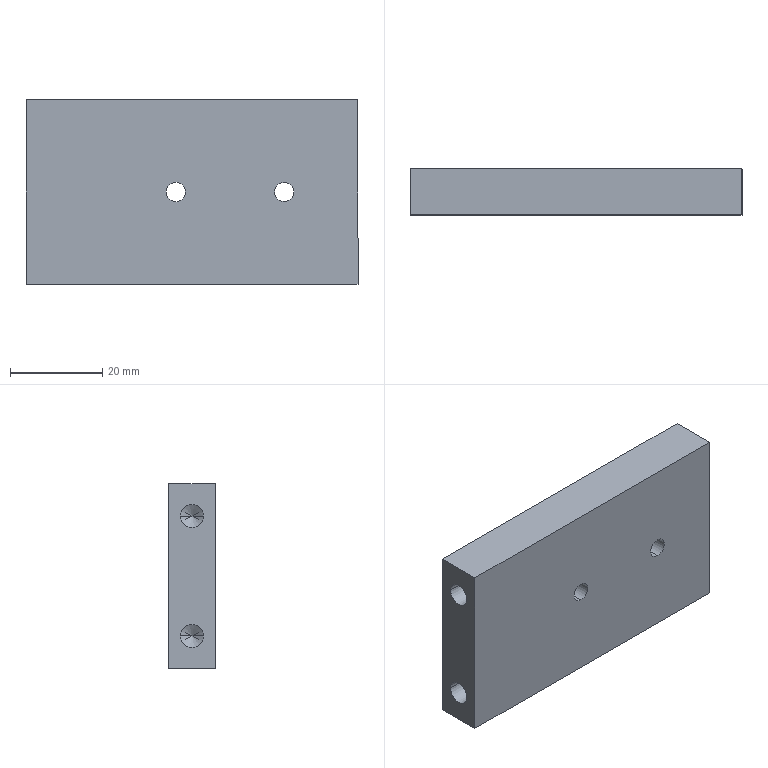Component | SolidWorks | SL021-102-4074.SL4PRT-1 | 1 solid | 18 faces | box 72 x 10 x 40 mm | volume 27718 mm3 | cylinder 8 | plane 6 | cone 4 | commonest cylinder face diameters 4.2 x4 5 x4 | material AL6061
build123d program:
from build123d import *

# Parameters (mm, degrees)
SKETCH1_W             = 40
SKETCH1_H             = 72
BOSS_EXTRUDE1_DEPTH   = 5
M6_TAPPED_HOLE1_D     = 5
M6_TAPPED_HOLE1_DEPTH = 20
M6_TAPPED_HOLE1_TIP   = 1.502
M5_TAPPED_HOLE1_D     = 4.2


with BuildPart() as part:
    # Sketch1 → Boss-Extrude1 (new, symmetric)
    with BuildSketch(Plane.XY):
        Rectangle(SKETCH1_W, SKETCH1_H)
    extrude(amount=BOSS_EXTRUDE1_DEPTH, both=True)

    # M6 Tapped Hole1
    with Locations(Plane(origin=(0, -36, -55), x_dir=(1, 0, 0), z_dir=(0, -1, 0))):
        with Locations((-13, 55), (13, 55)):
            Hole(M6_TAPPED_HOLE1_D / 2, depth=M6_TAPPED_HOLE1_DEPTH)
            with Locations((0, 0, -(M6_TAPPED_HOLE1_DEPTH + M6_TAPPED_HOLE1_TIP / 2))):  # 118° drill point
                Cone(0, M6_TAPPED_HOLE1_D / 2, M6_TAPPED_HOLE1_TIP, mode=Mode.SUBTRACT)

    # M5 Tapped Hole1 (through all)
    with Locations(Plane.XY.offset(5)):
        with Locations((0, 20), (0, -3.5)):
            Hole(M5_TAPPED_HOLE1_D / 2)


solid = part.part

# Placed as in the assembly
solid = solid.moved(Location((71.837, 179.501, -198.378), (90, 0, -90)))
STEP:
#1=COLOUR_RGB('',0.7922,0.8196,0.9333);
#2=FILL_AREA_STYLE_COLOUR('',#1);
#3=FILL_AREA_STYLE('',(#2));
#4=SURFACE_STYLE_FILL_AREA(#3);
#5=SURFACE_SIDE_STYLE('',(#4));
#6=SURFACE_STYLE_USAGE(.BOTH.,#5);
#7=PRESENTATION_STYLE_ASSIGNMENT((#6));
#8=CARTESIAN_POINT('',(3.616,6.87,-7.893));
#9=VERTEX_POINT('',#8);
#10=CARTESIAN_POINT('',(3.616,6.87,-7.727));
#11=VERTEX_POINT('',#10);
#12=CARTESIAN_POINT('',(3.616,6.87,-7.81));
#13=DIRECTION('',(0.,1.,0.));
#14=DIRECTION('',(0.,0.,1.));
#15=AXIS2_PLACEMENT_3D('',#12,#13,#14);
#16=CIRCLE('',#15,0.08268);
#17=EDGE_CURVE('',#9,#11,#16,.T.);
#18=ORIENTED_EDGE('',*,*,#17,.F.);
#19=CARTESIAN_POINT('',(3.616,7.264,-7.893));
#20=VERTEX_POINT('',#19);
#21=CARTESIAN_POINT('',(3.616,7.264,-7.893));
#22=DIRECTION('',(0.,1.,0.));
#23=VECTOR('',#22,39.37);
#24=LINE('',#21,#23);
#25=EDGE_CURVE('',#9,#20,#24,.T.);
#26=ORIENTED_EDGE('',*,*,#25,.T.);
#27=CARTESIAN_POINT('',(3.616,7.264,-7.727));
#28=VERTEX_POINT('',#27);
#29=CARTESIAN_POINT('',(3.616,7.264,-7.81));
#30=DIRECTION('',(0.,1.,0.));
#31=DIRECTION('',(0.,0.,1.));
#32=AXIS2_PLACEMENT_3D('',#29,#30,#31);
#33=CIRCLE('',#32,0.08268);
#34=EDGE_CURVE('',#20,#28,#33,.T.);
#35=ORIENTED_EDGE('',*,*,#34,.T.);
#36=CARTESIAN_POINT('',(3.616,7.264,-7.727));
#37=DIRECTION('',(0.,1.,0.));
#38=VECTOR('',#37,39.37);
#39=LINE('',#36,#38);
#40=EDGE_CURVE('',#11,#28,#39,.T.);
#41=ORIENTED_EDGE('',*,*,#40,.F.);
#42=EDGE_LOOP('',(#18,#26,#35,#41));
#43=FACE_OUTER_BOUND('',#42,.T.);
#44=CARTESIAN_POINT('',(3.616,7.264,-7.81));
#45=DIRECTION('',(0.,1.,0.));
#46=DIRECTION('',(0.,0.,1.));
#47=AXIS2_PLACEMENT_3D('',#44,#45,#46);
#48=CYLINDRICAL_SURFACE('',#47,0.08268);
#49=ADVANCED_FACE('',(#43),#48,.F.);
#50=CARTESIAN_POINT('',(2.69,6.87,-7.893));
#51=VERTEX_POINT('',#50);
#52=CARTESIAN_POINT('',(2.69,6.87,-7.727));
#53=VERTEX_POINT('',#52);
#54=CARTESIAN_POINT('',(2.69,6.87,-7.81));
#55=DIRECTION('',(0.,1.,0.));
#56=DIRECTION('',(0.,0.,1.));
#57=AXIS2_PLACEMENT_3D('',#54,#55,#56);
#58=CIRCLE('',#57,0.08268);
#59=EDGE_CURVE('',#51,#53,#58,.T.);
#60=ORIENTED_EDGE('',*,*,#59,.F.);
#61=CARTESIAN_POINT('',(2.69,7.264,-7.893));
#62=VERTEX_POINT('',#61);
#63=CARTESIAN_POINT('',(2.69,7.264,-7.893));
#64=DIRECTION('',(0.,1.,0.));
#65=VECTOR('',#64,39.37);
#66=LINE('',#63,#65);
#67=EDGE_CURVE('',#51,#62,#66,.T.);
#68=ORIENTED_EDGE('',*,*,#67,.T.);
#69=CARTESIAN_POINT('',(2.69,7.264,-7.727));
#70=VERTEX_POINT('',#69);
#71=CARTESIAN_POINT('',(2.69,7.264,-7.81));
#72=DIRECTION('',(0.,1.,0.));
#73=DIRECTION('',(0.,0.,1.));
#74=AXIS2_PLACEMENT_3D('',#71,#72,#73);
#75=CIRCLE('',#74,0.08268);
#76=EDGE_CURVE('',#62,#70,#75,.T.);
#77=ORIENTED_EDGE('',*,*,#76,.T.);
#78=CARTESIAN_POINT('',(2.69,7.264,-7.727));
#79=DIRECTION('',(0.,1.,0.));
#80=VECTOR('',#79,39.37);
#81=LINE('',#78,#80);
#82=EDGE_CURVE('',#53,#70,#81,.T.);
#83=ORIENTED_EDGE('',*,*,#82,.F.);
#84=EDGE_LOOP('',(#60,#68,#77,#83));
#85=FACE_OUTER_BOUND('',#84,.T.);
#86=CARTESIAN_POINT('',(2.69,7.264,-7.81));
#87=DIRECTION('',(0.,1.,0.));
#88=DIRECTION('',(0.,0.,1.));
#89=AXIS2_PLACEMENT_3D('',#86,#87,#88);
#90=CYLINDRICAL_SURFACE('',#89,0.08268);
#91=ADVANCED_FACE('',(#85),#90,.F.);
#92=CARTESIAN_POINT('',(2.198,7.165,-8.322));
#93=VERTEX_POINT('',#92);
#94=CARTESIAN_POINT('',(2.198,6.969,-8.322));
#95=VERTEX_POINT('',#94);
#96=CARTESIAN_POINT('',(2.198,7.067,-8.322));
#97=DIRECTION('',(-1.,0.,-0.));
#98=DIRECTION('',(0.,-1.,0.));
#99=AXIS2_PLACEMENT_3D('',#96,#97,#98);
#100=CIRCLE('',#99,0.09843);
#101=EDGE_CURVE('',#93,#95,#100,.T.);
#102=ORIENTED_EDGE('',*,*,#101,.F.);
#103=CARTESIAN_POINT('',(1.411,7.165,-8.322));
#104=VERTEX_POINT('',#103);
#105=CARTESIAN_POINT('',(1.411,7.165,-8.322));
#106=DIRECTION('',(-1.,0.,-0.));
#107=VECTOR('',#106,39.37);
#108=LINE('',#105,#107);
#109=EDGE_CURVE('',#93,#104,#108,.T.);
#110=ORIENTED_EDGE('',*,*,#109,.T.);
#111=CARTESIAN_POINT('',(1.411,6.969,-8.322));
#112=VERTEX_POINT('',#111);
#113=CARTESIAN_POINT('',(1.411,7.067,-8.322));
#114=DIRECTION('',(-1.,0.,-0.));
#115=DIRECTION('',(0.,-1.,0.));
#116=AXIS2_PLACEMENT_3D('',#113,#114,#115);
#117=CIRCLE('',#116,0.09843);
#118=EDGE_CURVE('',#104,#112,#117,.T.);
#119=ORIENTED_EDGE('',*,*,#118,.T.);
#120=CARTESIAN_POINT('',(1.411,6.969,-8.322));
#121=DIRECTION('',(-1.,0.,-0.));
#122=VECTOR('',#121,39.37);
#123=LINE('',#120,#122);
#124=EDGE_CURVE('',#95,#112,#123,.T.);
#125=ORIENTED_EDGE('',*,*,#124,.F.);
#126=EDGE_LOOP('',(#102,#110,#119,#125));
#127=FACE_OUTER_BOUND('',#126,.T.);
#128=CARTESIAN_POINT('',(1.411,7.067,-8.322));
#129=DIRECTION('',(-1.,0.,-0.));
#130=DIRECTION('',(0.,-1.,0.));
#131=AXIS2_PLACEMENT_3D('',#128,#129,#130);
#132=CYLINDRICAL_SURFACE('',#131,0.09843);
#133=ADVANCED_FACE('',(#127),#132,.F.);
#134=CARTESIAN_POINT('',(2.257,7.067,-8.322));
#135=VERTEX_POINT('',#134);
#136=CARTESIAN_POINT('',(2.198,6.969,-8.322));
#137=DIRECTION('',(-0.515,-0.8572,-0.));
#138=VECTOR('',#137,39.37);
#139=LINE('',#136,#138);
#140=EDGE_CURVE('',#135,#95,#139,.T.);
#141=ORIENTED_EDGE('',*,*,#140,.F.);
#142=CARTESIAN_POINT('',(2.198,7.165,-8.322));
#143=DIRECTION('',(-0.515,0.8572,0.));
#144=VECTOR('',#143,39.37);
#145=LINE('',#142,#144);
#146=EDGE_CURVE('',#135,#93,#145,.T.);
#147=ORIENTED_EDGE('',*,*,#146,.T.);
#148=ORIENTED_EDGE('',*,*,#101,.T.);
#149=EDGE_LOOP('',(#141,#147,#148));
#150=FACE_OUTER_BOUND('',#149,.T.);
#151=CARTESIAN_POINT('',(2.198,7.067,-8.322));
#152=DIRECTION('',(-1.,0.,-0.));
#153=DIRECTION('',(0.,-1.,0.));
#154=AXIS2_PLACEMENT_3D('',#151,#152,#153);
#155=CONICAL_SURFACE('',#154,0.09843,1.03);
#156=ADVANCED_FACE('',(#150),#155,.F.);
#157=CARTESIAN_POINT('',(2.198,7.165,-7.298));
#158=VERTEX_POINT('',#157);
#159=CARTESIAN_POINT('',(2.198,6.969,-7.298));
#160=VERTEX_POINT('',#159);
#161=CARTESIAN_POINT('',(2.198,7.067,-7.298));
#162=DIRECTION('',(-1.,0.,-0.));
#163=DIRECTION('',(0.,-1.,0.));
#164=AXIS2_PLACEMENT_3D('',#161,#162,#163);
#165=CIRCLE('',#164,0.09843);
#166=EDGE_CURVE('',#158,#160,#165,.T.);
#167=ORIENTED_EDGE('',*,*,#166,.F.);
#168=CARTESIAN_POINT('',(1.411,7.165,-7.298));
#169=VERTEX_POINT('',#168);
#170=CARTESIAN_POINT('',(1.411,7.165,-7.298));
#171=DIRECTION('',(-1.,0.,-0.));
#172=VECTOR('',#171,39.37);
#173=LINE('',#170,#172);
#174=EDGE_CURVE('',#158,#169,#173,.T.);
#175=ORIENTED_EDGE('',*,*,#174,.T.);
#176=CARTESIAN_POINT('',(1.411,6.969,-7.298));
#177=VERTEX_POINT('',#176);
#178=CARTESIAN_POINT('',(1.411,7.067,-7.298));
#179=DIRECTION('',(-1.,0.,-0.));
#180=DIRECTION('',(0.,-1.,0.));
#181=AXIS2_PLACEMENT_3D('',#178,#179,#180);
#182=CIRCLE('',#181,0.09843);
#183=EDGE_CURVE('',#169,#177,#182,.T.);
#184=ORIENTED_EDGE('',*,*,#183,.T.);
#185=CARTESIAN_POINT('',(1.411,6.969,-7.298));
#186=DIRECTION('',(-1.,0.,-0.));
#187=VECTOR('',#186,39.37);
#188=LINE('',#185,#187);
#189=EDGE_CURVE('',#160,#177,#188,.T.);
#190=ORIENTED_EDGE('',*,*,#189,.F.);
#191=EDGE_LOOP('',(#167,#175,#184,#190));
#192=FACE_OUTER_BOUND('',#191,.T.);
#193=CARTESIAN_POINT('',(1.411,7.067,-7.298));
#194=DIRECTION('',(-1.,0.,-0.));
#195=DIRECTION('',(0.,-1.,0.));
#196=AXIS2_PLACEMENT_3D('',#193,#194,#195);
#197=CYLINDRICAL_SURFACE('',#196,0.09843);
#198=ADVANCED_FACE('',(#192),#197,.F.);
#199=CARTESIAN_POINT('',(2.257,7.067,-7.298));
#200=VERTEX_POINT('',#199);
#201=CARTESIAN_POINT('',(2.198,6.969,-7.298));
#202=DIRECTION('',(-0.515,-0.8572,-0.));
#203=VECTOR('',#202,39.37);
#204=LINE('',#201,#203);
#205=EDGE_CURVE('',#200,#160,#204,.T.);
#206=ORIENTED_EDGE('',*,*,#205,.F.);
#207=CARTESIAN_POINT('',(2.198,7.165,-7.298));
#208=DIRECTION('',(-0.515,0.8572,0.));
#209=VECTOR('',#208,39.37);
#210=LINE('',#207,#209);
#211=EDGE_CURVE('',#200,#158,#210,.T.);
#212=ORIENTED_EDGE('',*,*,#211,.T.);
#213=ORIENTED_EDGE('',*,*,#166,.T.);
#214=EDGE_LOOP('',(#206,#212,#213));
#215=FACE_OUTER_BOUND('',#214,.T.);
#216=CARTESIAN_POINT('',(2.198,7.067,-7.298));
#217=DIRECTION('',(-1.,0.,-0.));
#218=DIRECTION('',(0.,-1.,0.));
#219=AXIS2_PLACEMENT_3D('',#216,#217,#218);
#220=CONICAL_SURFACE('',#219,0.09843,1.03);
#221=ADVANCED_FACE('',(#215),#220,.F.);
#222=CARTESIAN_POINT('',(1.411,6.87,-7.023));
#223=VERTEX_POINT('',#222);
#224=CARTESIAN_POINT('',(4.246,6.87,-7.023));
#225=VERTEX_POINT('',#224);
#226=CARTESIAN_POINT('',(1.411,6.87,-7.023));
#227=DIRECTION('',(1.,-0.,0.));
#228=VECTOR('',#227,39.37);
#229=LINE('',#226,#228);
#230=EDGE_CURVE('',#223,#225,#229,.T.);
#231=ORIENTED_EDGE('',*,*,#230,.T.);
#232=CARTESIAN_POINT('',(4.246,7.264,-7.023));
#233=VERTEX_POINT('',#232);
#234=CARTESIAN_POINT('',(4.246,7.264,-7.023));
#235=DIRECTION('',(-0.,-1.,-0.));
#236=VECTOR('',#235,39.37);
#237=LINE('',#234,#236);
#238=EDGE_CURVE('',#233,#225,#237,.T.);
#239=ORIENTED_EDGE('',*,*,#238,.F.);
#240=CARTESIAN_POINT('',(1.411,7.264,-7.023));
#241=VERTEX_POINT('',#240);
#242=CARTESIAN_POINT('',(1.411,7.264,-7.023));
#243=DIRECTION('',(1.,-0.,0.));
#244=VECTOR('',#243,39.37);
#245=LINE('',#242,#244);
#246=EDGE_CURVE('',#241,#233,#245,.T.);
#247=ORIENTED_EDGE('',*,*,#246,.F.);
#248=CARTESIAN_POINT('',(1.411,7.264,-7.023));
#249=DIRECTION('',(-0.,-1.,-0.));
#250=VECTOR('',#249,39.37);
#251=LINE('',#248,#250);
#252=EDGE_CURVE('',#241,#223,#251,.T.);
#253=ORIENTED_EDGE('',*,*,#252,.T.);
#254=EDGE_LOOP('',(#231,#239,#247,#253));
#255=FACE_OUTER_BOUND('',#254,.T.);
#256=CARTESIAN_POINT('',(1.411,7.264,-7.023));
#257=DIRECTION('',(0.,0.,-1.));
#258=DIRECTION('',(0.,1.,0.));
#259=AXIS2_PLACEMENT_3D('',#256,#257,#258);
#260=PLANE('',#259);
#261=ADVANCED_FACE('',(#255),#260,.F.);
#262=CARTESIAN_POINT('',(4.246,6.87,-8.598));
#263=VERTEX_POINT('',#262);
#264=CARTESIAN_POINT('',(4.246,6.87,-8.598));
#265=DIRECTION('',(0.,0.,-1.));
#266=VECTOR('',#265,39.37);
#267=LINE('',#264,#266);
#268=EDGE_CURVE('',#225,#263,#267,.T.);
#269=ORIENTED_EDGE('',*,*,#268,.T.);
#270=CARTESIAN_POINT('',(4.246,7.264,-8.598));
#271=VERTEX_POINT('',#270);
#272=CARTESIAN_POINT('',(4.246,7.264,-8.598));
#273=DIRECTION('',(-0.,-1.,-0.));
#274=VECTOR('',#273,39.37);
#275=LINE('',#272,#274);
#276=EDGE_CURVE('',#271,#263,#275,.T.);
#277=ORIENTED_EDGE('',*,*,#276,.F.);
#278=CARTESIAN_POINT('',(4.246,7.264,-8.598));
#279=DIRECTION('',(0.,0.,-1.));
#280=VECTOR('',#279,39.37);
#281=LINE('',#278,#280);
#282=EDGE_CURVE('',#233,#271,#281,.T.);
#283=ORIENTED_EDGE('',*,*,#282,.F.);
#284=ORIENTED_EDGE('',*,*,#238,.T.);
#285=EDGE_LOOP('',(#269,#277,#283,#284));
#286=FACE_OUTER_BOUND('',#285,.T.);
#287=CARTESIAN_POINT('',(4.246,7.264,-8.598));
#288=DIRECTION('',(-1.,0.,-0.));
#289=DIRECTION('',(-0.,-1.,-0.));
#290=AXIS2_PLACEMENT_3D('',#287,#288,#289);
#291=PLANE('',#290);
#292=ADVANCED_FACE('',(#286),#291,.F.);
#293=CARTESIAN_POINT('',(1.411,6.87,-8.598));
#294=VERTEX_POINT('',#293);
#295=CARTESIAN_POINT('',(1.411,6.87,-8.598));
#296=DIRECTION('',(-1.,0.,-0.));
#297=VECTOR('',#296,39.37);
#298=LINE('',#295,#297);
#299=EDGE_CURVE('',#263,#294,#298,.T.);
#300=ORIENTED_EDGE('',*,*,#299,.T.);
#301=CARTESIAN_POINT('',(1.411,7.264,-8.598));
#302=VERTEX_POINT('',#301);
#303=CARTESIAN_POINT('',(1.411,7.264,-8.598));
#304=DIRECTION('',(-0.,-1.,-0.));
#305=VECTOR('',#304,39.37);
#306=LINE('',#303,#305);
#307=EDGE_CURVE('',#302,#294,#306,.T.);
#308=ORIENTED_EDGE('',*,*,#307,.F.);
#309=CARTESIAN_POINT('',(1.411,7.264,-8.598));
#310=DIRECTION('',(-1.,0.,-0.));
#311=VECTOR('',#310,39.37);
#312=LINE('',#309,#311);
#313=EDGE_CURVE('',#271,#302,#312,.T.);
#314=ORIENTED_EDGE('',*,*,#313,.F.);
#315=ORIENTED_EDGE('',*,*,#276,.T.);
#316=EDGE_LOOP('',(#300,#308,#314,#315));
#317=FACE_OUTER_BOUND('',#316,.T.);
#318=CARTESIAN_POINT('',(1.411,7.264,-8.598));
#319=DIRECTION('',(-0.,-0.,1.));
#320=DIRECTION('',(-0.,-1.,-0.));
#321=AXIS2_PLACEMENT_3D('',#318,#319,#320);
#322=PLANE('',#321);
#323=ADVANCED_FACE('',(#317),#322,.F.);
#324=CARTESIAN_POINT('',(1.411,7.067,-8.322));
#325=DIRECTION('',(-1.,0.,-0.));
#326=DIRECTION('',(0.,-1.,0.));
#327=AXIS2_PLACEMENT_3D('',#324,#325,#326);
#328=CIRCLE('',#327,0.09843);
#329=EDGE_CURVE('',#112,#104,#328,.T.);
#330=ORIENTED_EDGE('',*,*,#329,.F.);
#331=ORIENTED_EDGE('',*,*,#118,.F.);
#332=EDGE_LOOP('',(#330,#331));
#333=FACE_BOUND('',#332,.T.);
#334=CARTESIAN_POINT('',(1.411,7.067,-7.298));
#335=DIRECTION('',(-1.,0.,-0.));
#336=DIRECTION('',(0.,-1.,0.));
#337=AXIS2_PLACEMENT_3D('',#334,#335,#336);
#338=CIRCLE('',#337,0.09843);
#339=EDGE_CURVE('',#177,#169,#338,.T.);
#340=ORIENTED_EDGE('',*,*,#339,.F.);
#341=ORIENTED_EDGE('',*,*,#183,.F.);
#342=EDGE_LOOP('',(#340,#341));
#343=FACE_BOUND('',#342,.T.);
#344=CARTESIAN_POINT('',(1.411,6.87,-8.598));
#345=DIRECTION('',(-0.,-0.,1.));
#346=VECTOR('',#345,39.37);
#347=LINE('',#344,#346);
#348=EDGE_CURVE('',#294,#223,#347,.T.);
#349=ORIENTED_EDGE('',*,*,#348,.T.);
#350=ORIENTED_EDGE('',*,*,#252,.F.);
#351=CARTESIAN_POINT('',(1.411,7.264,-8.598));
#352=DIRECTION('',(-0.,-0.,1.));
#353=VECTOR('',#352,39.37);
#354=LINE('',#351,#353);
#355=EDGE_CURVE('',#302,#241,#354,.T.);
#356=ORIENTED_EDGE('',*,*,#355,.F.);
#357=ORIENTED_EDGE('',*,*,#307,.T.);
#358=EDGE_LOOP('',(#349,#350,#356,#357));
#359=FACE_OUTER_BOUND('',#358,.T.);
#360=CARTESIAN_POINT('',(1.411,7.264,-8.598));
#361=DIRECTION('',(1.,-0.,0.));
#362=DIRECTION('',(0.,1.,0.));
#363=AXIS2_PLACEMENT_3D('',#360,#361,#362);
#364=PLANE('',#363);
#365=ADVANCED_FACE('',(#333,#343,#359),#364,.F.);
#366=CARTESIAN_POINT('',(3.616,7.264,-7.81));
#367=DIRECTION('',(0.,1.,0.));
#368=DIRECTION('',(0.,0.,1.));
#369=AXIS2_PLACEMENT_3D('',#366,#367,#368);
#370=CIRCLE('',#369,0.08268);
#371=EDGE_CURVE('',#28,#20,#370,.T.);
#372=ORIENTED_EDGE('',*,*,#371,.F.);
#373=ORIENTED_EDGE('',*,*,#34,.F.);
#374=EDGE_LOOP('',(#372,#373));
#375=FACE_BOUND('',#374,.T.);
#376=CARTESIAN_POINT('',(2.69,7.264,-7.81));
#377=DIRECTION('',(0.,1.,0.));
#378=DIRECTION('',(0.,0.,1.));
#379=AXIS2_PLACEMENT_3D('',#376,#377,#378);
#380=CIRCLE('',#379,0.08268);
#381=EDGE_CURVE('',#70,#62,#380,.T.);
#382=ORIENTED_EDGE('',*,*,#381,.F.);
#383=ORIENTED_EDGE('',*,*,#76,.F.);
#384=EDGE_LOOP('',(#382,#383));
#385=FACE_BOUND('',#384,.T.);
#386=ORIENTED_EDGE('',*,*,#246,.T.);
#387=ORIENTED_EDGE('',*,*,#282,.T.);
#388=ORIENTED_EDGE('',*,*,#313,.T.);
#389=ORIENTED_EDGE('',*,*,#355,.T.);
#390=EDGE_LOOP('',(#386,#387,#388,#389));
#391=FACE_OUTER_BOUND('',#390,.T.);
#392=CARTESIAN_POINT('',(2.828,7.264,-7.81));
#393=DIRECTION('',(-0.,-1.,-0.));
#394=DIRECTION('',(0.,0.,-1.));
#395=AXIS2_PLACEMENT_3D('',#392,#393,#394);
#396=PLANE('',#395);
#397=ADVANCED_FACE('',(#375,#385,#391),#396,.F.);
#398=CARTESIAN_POINT('',(3.616,6.87,-7.81));
#399=DIRECTION('',(0.,1.,0.));
#400=DIRECTION('',(0.,0.,1.));
#401=AXIS2_PLACEMENT_3D('',#398,#399,#400);
#402=CIRCLE('',#401,0.08268);
#403=EDGE_CURVE('',#11,#9,#402,.T.);
#404=ORIENTED_EDGE('',*,*,#403,.T.);
#405=ORIENTED_EDGE('',*,*,#17,.T.);
#406=EDGE_LOOP('',(#404,#405));
#407=FACE_BOUND('',#406,.T.);
#408=CARTESIAN_POINT('',(2.69,6.87,-7.81));
#409=DIRECTION('',(0.,1.,0.));
#410=DIRECTION('',(0.,0.,1.));
#411=AXIS2_PLACEMENT_3D('',#408,#409,#410);
#412=CIRCLE('',#411,0.08268);
#413=EDGE_CURVE('',#53,#51,#412,.T.);
#414=ORIENTED_EDGE('',*,*,#413,.T.);
#415=ORIENTED_EDGE('',*,*,#59,.T.);
#416=EDGE_LOOP('',(#414,#415));
#417=FACE_BOUND('',#416,.T.);
#418=ORIENTED_EDGE('',*,*,#230,.F.);
#419=ORIENTED_EDGE('',*,*,#348,.F.);
#420=ORIENTED_EDGE('',*,*,#299,.F.);
#421=ORIENTED_EDGE('',*,*,#268,.F.);
#422=EDGE_LOOP('',(#418,#419,#420,#421));
#423=FACE_OUTER_BOUND('',#422,.T.);
#424=CARTESIAN_POINT('',(2.828,6.87,-7.81));
#425=DIRECTION('',(-0.,-1.,-0.));
#426=DIRECTION('',(0.,0.,-1.));
#427=AXIS2_PLACEMENT_3D('',#424,#425,#426);
#428=PLANE('',#427);
#429=ADVANCED_FACE('',(#407,#417,#423),#428,.T.);
#430=ORIENTED_EDGE('',*,*,#211,.F.);
#431=ORIENTED_EDGE('',*,*,#205,.T.);
#432=CARTESIAN_POINT('',(2.198,7.067,-7.298));
#433=DIRECTION('',(-1.,0.,-0.));
#434=DIRECTION('',(0.,-1.,0.));
#435=AXIS2_PLACEMENT_3D('',#432,#433,#434);
#436=CIRCLE('',#435,0.09843);
#437=EDGE_CURVE('',#160,#158,#436,.T.);
#438=ORIENTED_EDGE('',*,*,#437,.T.);
#439=EDGE_LOOP('',(#430,#431,#438));
#440=FACE_OUTER_BOUND('',#439,.T.);
#441=CARTESIAN_POINT('',(2.198,7.067,-7.298));
#442=DIRECTION('',(-1.,0.,-0.));
#443=DIRECTION('',(0.,-1.,0.));
#444=AXIS2_PLACEMENT_3D('',#441,#442,#443);
#445=CONICAL_SURFACE('',#444,0.09843,1.03);
#446=ADVANCED_FACE('',(#440),#445,.F.);
#447=ORIENTED_EDGE('',*,*,#174,.F.);
#448=ORIENTED_EDGE('',*,*,#437,.F.);
#449=ORIENTED_EDGE('',*,*,#189,.T.);
#450=ORIENTED_EDGE('',*,*,#339,.T.);
#451=EDGE_LOOP('',(#447,#448,#449,#450));
#452=FACE_OUTER_BOUND('',#451,.T.);
#453=CARTESIAN_POINT('',(1.411,7.067,-7.298));
#454=DIRECTION('',(-1.,0.,-0.));
#455=DIRECTION('',(0.,-1.,0.));
#456=AXIS2_PLACEMENT_3D('',#453,#454,#455);
#457=CYLINDRICAL_SURFACE('',#456,0.09843);
#458=ADVANCED_FACE('',(#452),#457,.F.);
#459=ORIENTED_EDGE('',*,*,#146,.F.);
#460=ORIENTED_EDGE('',*,*,#140,.T.);
#461=CARTESIAN_POINT('',(2.198,7.067,-8.322));
#462=DIRECTION('',(-1.,0.,-0.));
#463=DIRECTION('',(0.,-1.,0.));
#464=AXIS2_PLACEMENT_3D('',#461,#462,#463);
#465=CIRCLE('',#464,0.09843);
#466=EDGE_CURVE('',#95,#93,#465,.T.);
#467=ORIENTED_EDGE('',*,*,#466,.T.);
#468=EDGE_LOOP('',(#459,#460,#467));
#469=FACE_OUTER_BOUND('',#468,.T.);
#470=CARTESIAN_POINT('',(2.198,7.067,-8.322));
#471=DIRECTION('',(-1.,0.,-0.));
#472=DIRECTION('',(0.,-1.,0.));
#473=AXIS2_PLACEMENT_3D('',#470,#471,#472);
#474=CONICAL_SURFACE('',#473,0.09843,1.03);
#475=ADVANCED_FACE('',(#469),#474,.F.);
#476=ORIENTED_EDGE('',*,*,#109,.F.);
#477=ORIENTED_EDGE('',*,*,#466,.F.);
#478=ORIENTED_EDGE('',*,*,#124,.T.);
#479=ORIENTED_EDGE('',*,*,#329,.T.);
#480=EDGE_LOOP('',(#476,#477,#478,#479));
#481=FACE_OUTER_BOUND('',#480,.T.);
#482=CARTESIAN_POINT('',(1.411,7.067,-8.322));
#483=DIRECTION('',(-1.,0.,-0.));
#484=DIRECTION('',(0.,-1.,0.));
#485=AXIS2_PLACEMENT_3D('',#482,#483,#484);
#486=CYLINDRICAL_SURFACE('',#485,0.09843);
#487=ADVANCED_FACE('',(#481),#486,.F.);
#488=ORIENTED_EDGE('',*,*,#67,.F.);
#489=ORIENTED_EDGE('',*,*,#413,.F.);
#490=ORIENTED_EDGE('',*,*,#82,.T.);
#491=ORIENTED_EDGE('',*,*,#381,.T.);
#492=EDGE_LOOP('',(#488,#489,#490,#491));
#493=FACE_OUTER_BOUND('',#492,.T.);
#494=CARTESIAN_POINT('',(2.69,7.264,-7.81));
#495=DIRECTION('',(0.,1.,0.));
#496=DIRECTION('',(0.,0.,1.));
#497=AXIS2_PLACEMENT_3D('',#494,#495,#496);
#498=CYLINDRICAL_SURFACE('',#497,0.08268);
#499=ADVANCED_FACE('',(#493),#498,.F.);
#500=ORIENTED_EDGE('',*,*,#25,.F.);
#501=ORIENTED_EDGE('',*,*,#403,.F.);
#502=ORIENTED_EDGE('',*,*,#40,.T.);
#503=ORIENTED_EDGE('',*,*,#371,.T.);
#504=EDGE_LOOP('',(#500,#501,#502,#503));
#505=FACE_OUTER_BOUND('',#504,.T.);
#506=CARTESIAN_POINT('',(3.616,7.264,-7.81));
#507=DIRECTION('',(0.,1.,0.));
#508=DIRECTION('',(0.,0.,1.));
#509=AXIS2_PLACEMENT_3D('',#506,#507,#508);
#510=CYLINDRICAL_SURFACE('',#509,0.08268);
#511=ADVANCED_FACE('',(#505),#510,.F.);
#512=CLOSED_SHELL('',(#49,#91,#133,#156,#198,#221,#261,#292,#323,#365,#397,#429,#446,#458,#475,#487,#499,#511));
#513=MANIFOLD_SOLID_BREP('',#512);
#514=STYLED_ITEM('',(#7),#513);
#515=(LENGTH_UNIT()NAMED_UNIT(*)SI_UNIT($,.METRE.));
#516=LENGTH_MEASURE_WITH_UNIT(LENGTH_MEASURE(0.0254),#515);
#517=DIMENSIONAL_EXPONENTS(1.,0.,0.,0.,0.,0.,0.);
#518=(CONVERSION_BASED_UNIT('',#516)LENGTH_UNIT()NAMED_UNIT(#517));
#519=UNCERTAINTY_MEASURE_WITH_UNIT(LENGTH_MEASURE(0.00001),#518,'','');
#520=(NAMED_UNIT(*)PLANE_ANGLE_UNIT()SI_UNIT($,.RADIAN.));
#521=(NAMED_UNIT(*)SI_UNIT($,.STERADIAN.)SOLID_ANGLE_UNIT());
#522=(GEOMETRIC_REPRESENTATION_CONTEXT(3)GLOBAL_UNCERTAINTY_ASSIGNED_CONTEXT((#519))GLOBAL_UNIT_ASSIGNED_CONTEXT((#518,#520,#521))REPRESENTATION_CONTEXT('',''));
#523=MECHANICAL_DESIGN_GEOMETRIC_PRESENTATION_REPRESENTATION('',(#514),#522);
#524=CARTESIAN_POINT('',(0.,0.,0.));
#525=DIRECTION('',(0.,0.,1.));
#526=DIRECTION('',(1.,0.,0.));
#527=AXIS2_PLACEMENT_3D('',#524,#525,#526);
#528=(LENGTH_UNIT()NAMED_UNIT(*)SI_UNIT($,.METRE.));
#529=LENGTH_MEASURE_WITH_UNIT(LENGTH_MEASURE(0.0254),#528);
#530=DIMENSIONAL_EXPONENTS(1.,0.,0.,0.,0.,0.,0.);
#531=(CONVERSION_BASED_UNIT('',#529)LENGTH_UNIT()NAMED_UNIT(#530));
#532=UNCERTAINTY_MEASURE_WITH_UNIT(LENGTH_MEASURE(0.00001),#531,'','');
#533=(NAMED_UNIT(*)PLANE_ANGLE_UNIT()SI_UNIT($,.RADIAN.));
#534=(NAMED_UNIT(*)SI_UNIT($,.STERADIAN.)SOLID_ANGLE_UNIT());
#535=(GEOMETRIC_REPRESENTATION_CONTEXT(3)GLOBAL_UNCERTAINTY_ASSIGNED_CONTEXT((#532))GLOBAL_UNIT_ASSIGNED_CONTEXT((#531,#533,#534))REPRESENTATION_CONTEXT('',''));
#536=ADVANCED_BREP_SHAPE_REPRESENTATION('',(#513,#527),#535);
#537=PRESENTATION_LAYER_ASSIGNMENT('','',(#514));